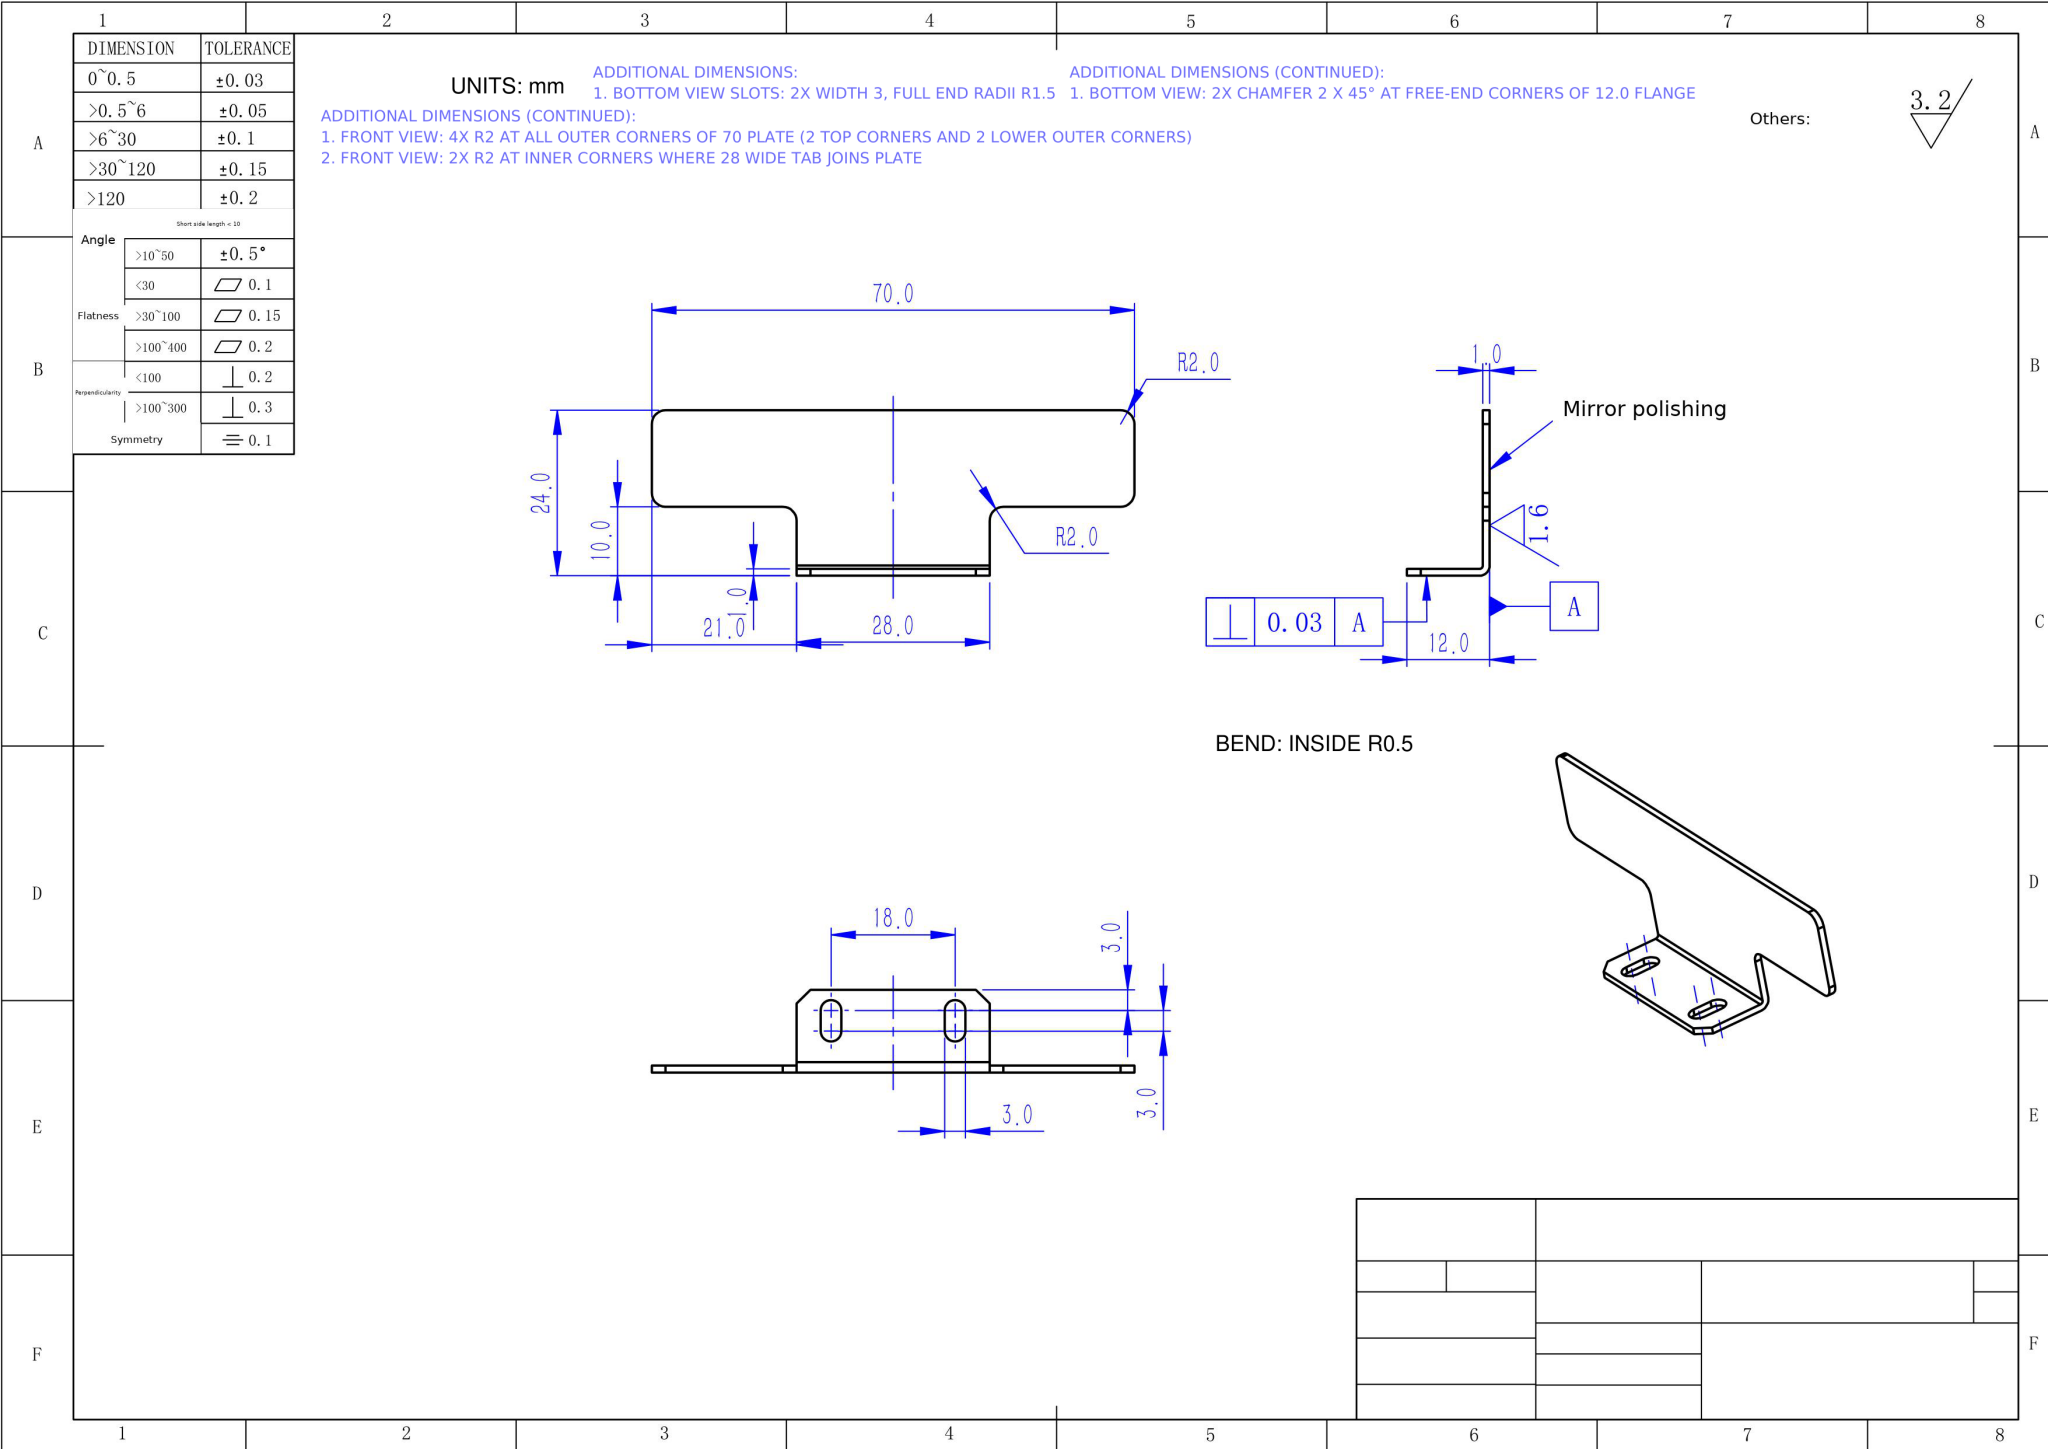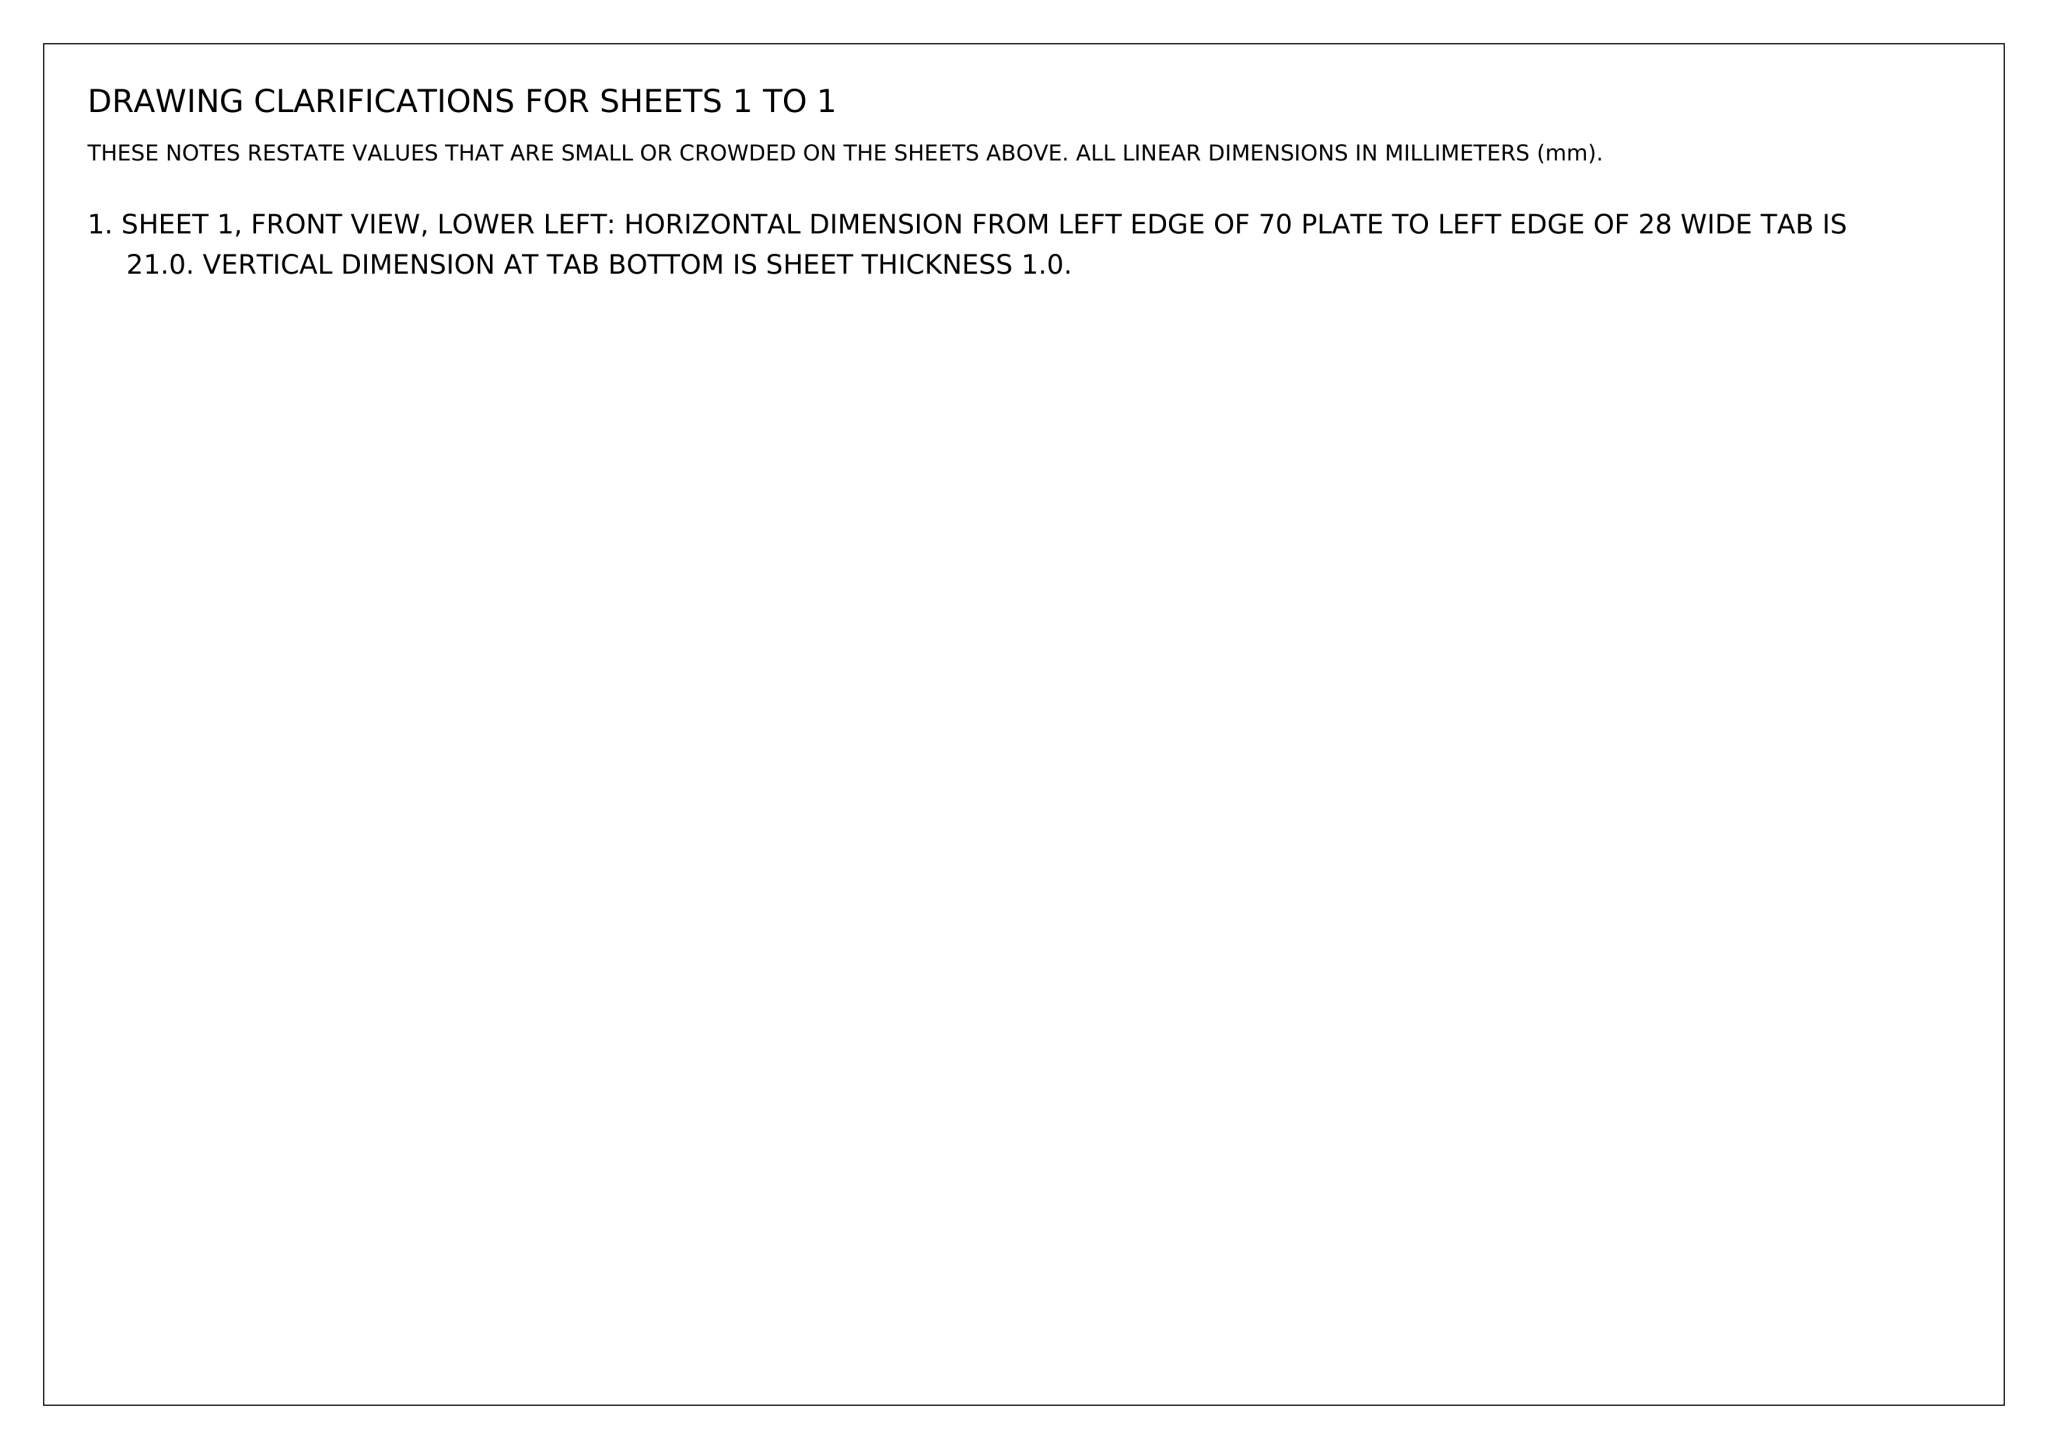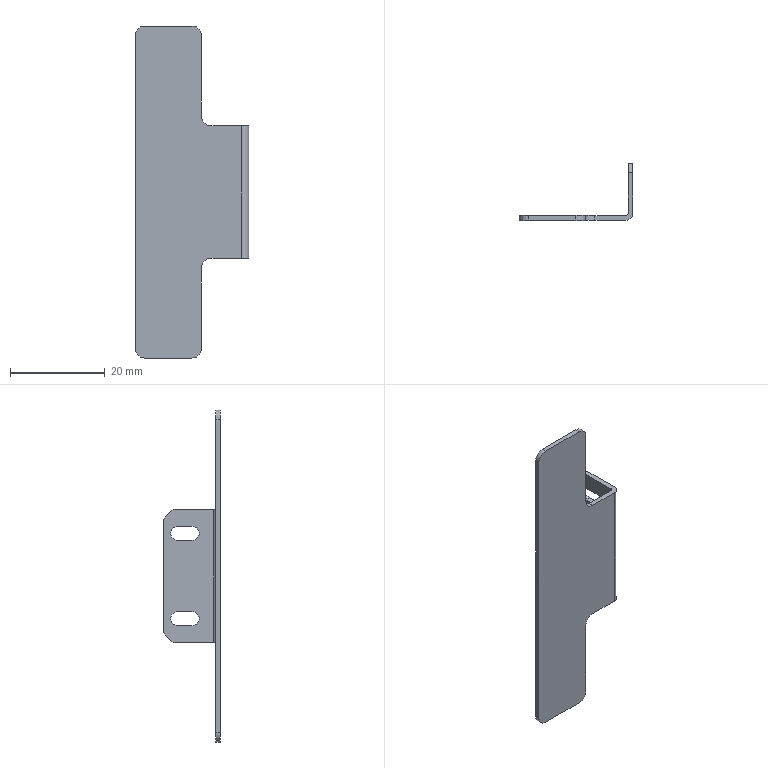Part | NX | mm | 1 solid | 30 faces | box 24 x 12 x 70 mm | volume 1518 mm3 | plane 18 | cylinder 12 | commonest cylinder face diameters 4 x6 3 x5 1 x1